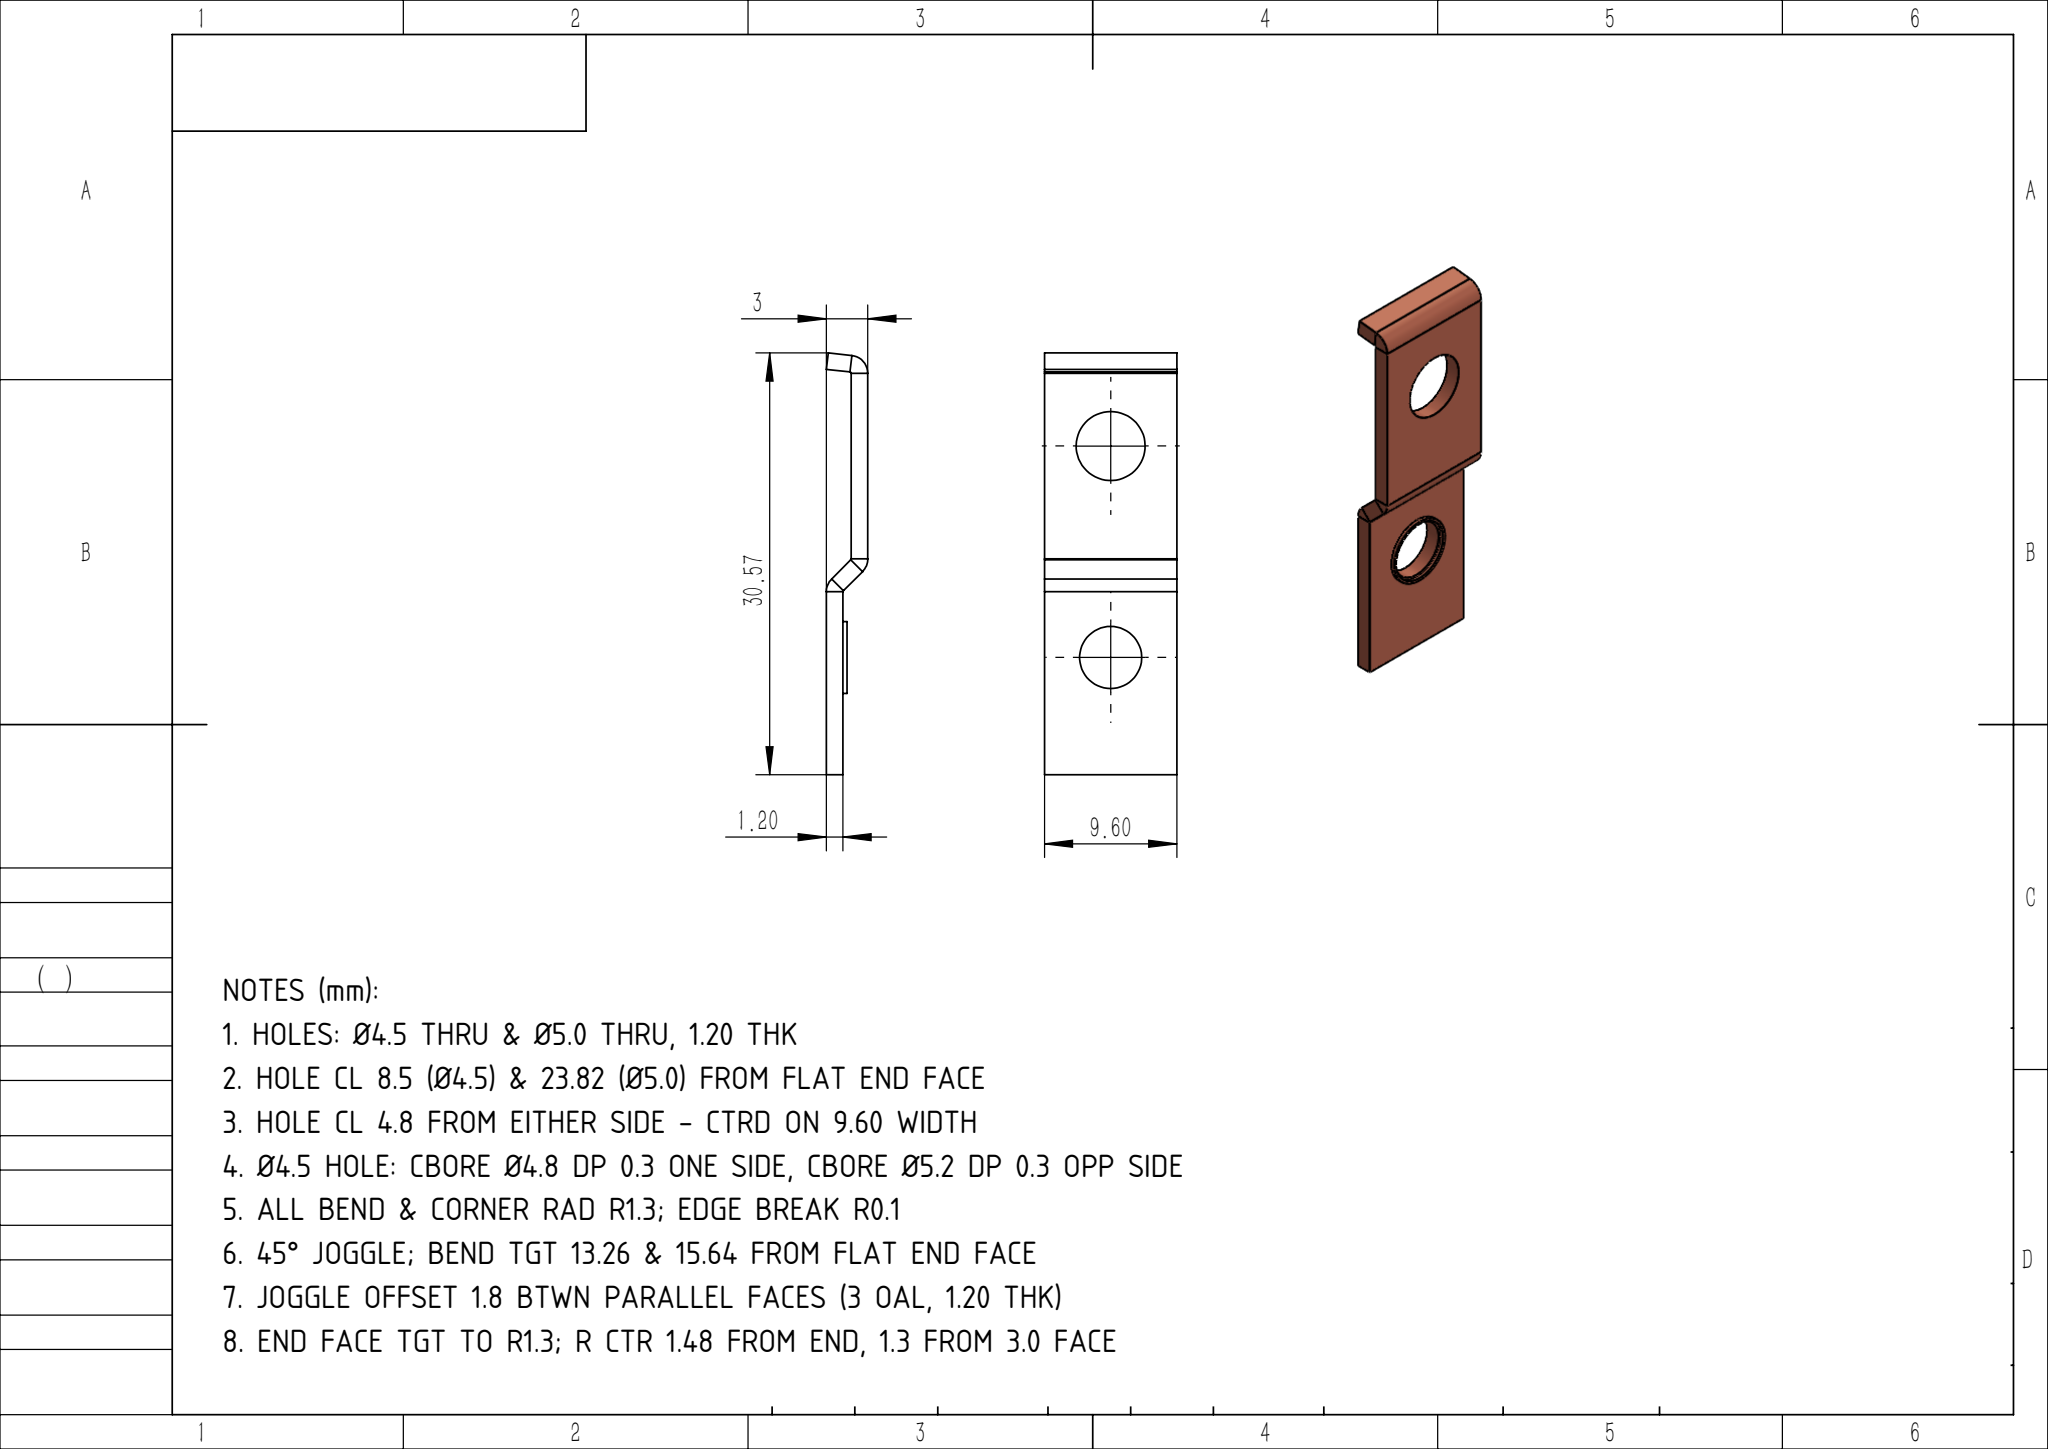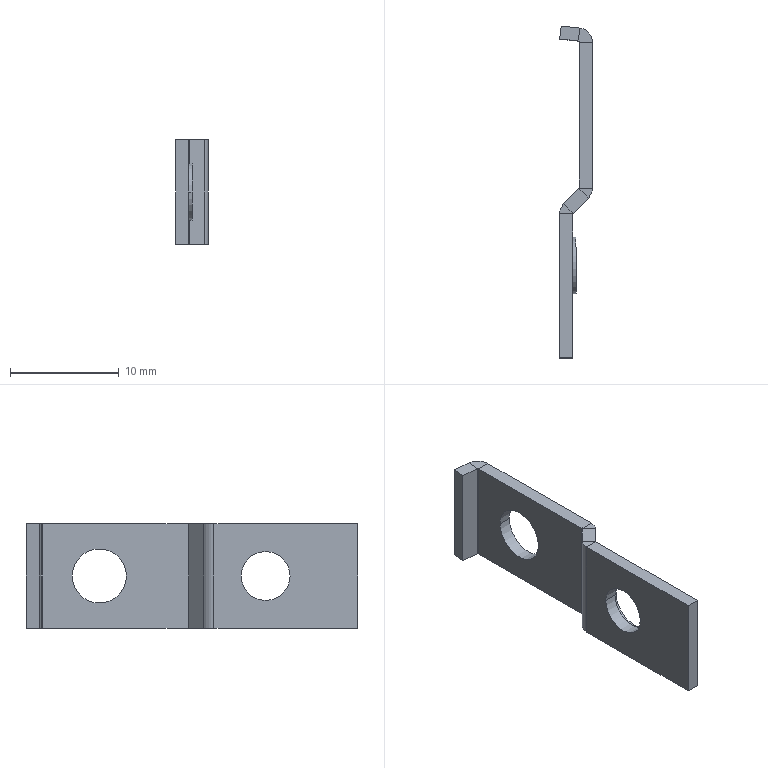Part | SolidWorks | mm | 1 solid | 40 faces | box 3 x 30.57 x 9.6 mm | volume 333 mm3 | plane 26 | cylinder 14 | commonest cylinder face diameters 0.2 x3 2.6 x3 4.8 x2 5.2 x2 4.5 x2 5 x2
Drawing notes:
HOLES: Ø4.5 THRU & Ø5.0 THRU, 1.20 THK | from the solid: cyl dia 4.5 axis x len 1.2 @ y=8.5; cyl dia 5.0 axis x len 1.2 @ y=23.82
HOLE CL 8.5 (Ø4.5) & 23.82 (Ø5.0) FROM FLAT END FACE | from the solid: hole axes at y=8.5 and y=23.82 from y=0 plane (only planar end face)
HOLE CL 4.8 FROM EITHER SIDE - CTRD ON 9.60 WIDTH | from the solid: both hole axes at z=4.8; z planes at 0 and 9.6
Ø4.5 HOLE: CBORE Ø4.8 DP 0.3 ONE SIDE, CBORE Ø5.2 DP 0.3 OPP SIDE | from the solid: cyl dia 4.8 len 0.3 and dia 5.2 len 0.3, both coaxial @ y=8.5, z=4.8
ALL BEND & CORNER RAD R1.3; EDGE BREAK R0.1 | from the solid: cyl dia 2.6 axis z at (1.3,13.26),(1.7,15.64),(1.7,29.09); dia 0.2 same axes
45° JOGGLE; BEND TGT 13.26 & 15.64 FROM FLAT END FACE | from the solid: R1.3 ctrs (x1.3,y13.26) tgt x=0 and (x1.7,y15.64) tgt x=3.0 give 45° incline
JOGGLE OFFSET 1.8 BTWN PARALLEL FACES (3 OAL, 1.20 THK) | from the solid: x planes 0/1.2 and 1.8/3.0; bbox x=3.0
END FACE TGT TO R1.3; R CTR 1.48 FROM END, 1.3 FROM 3.0 FACE | from the solid: R1.3 ctr (x1.7,y29.09), bbox y max 30.572, no planar face at y=30.572